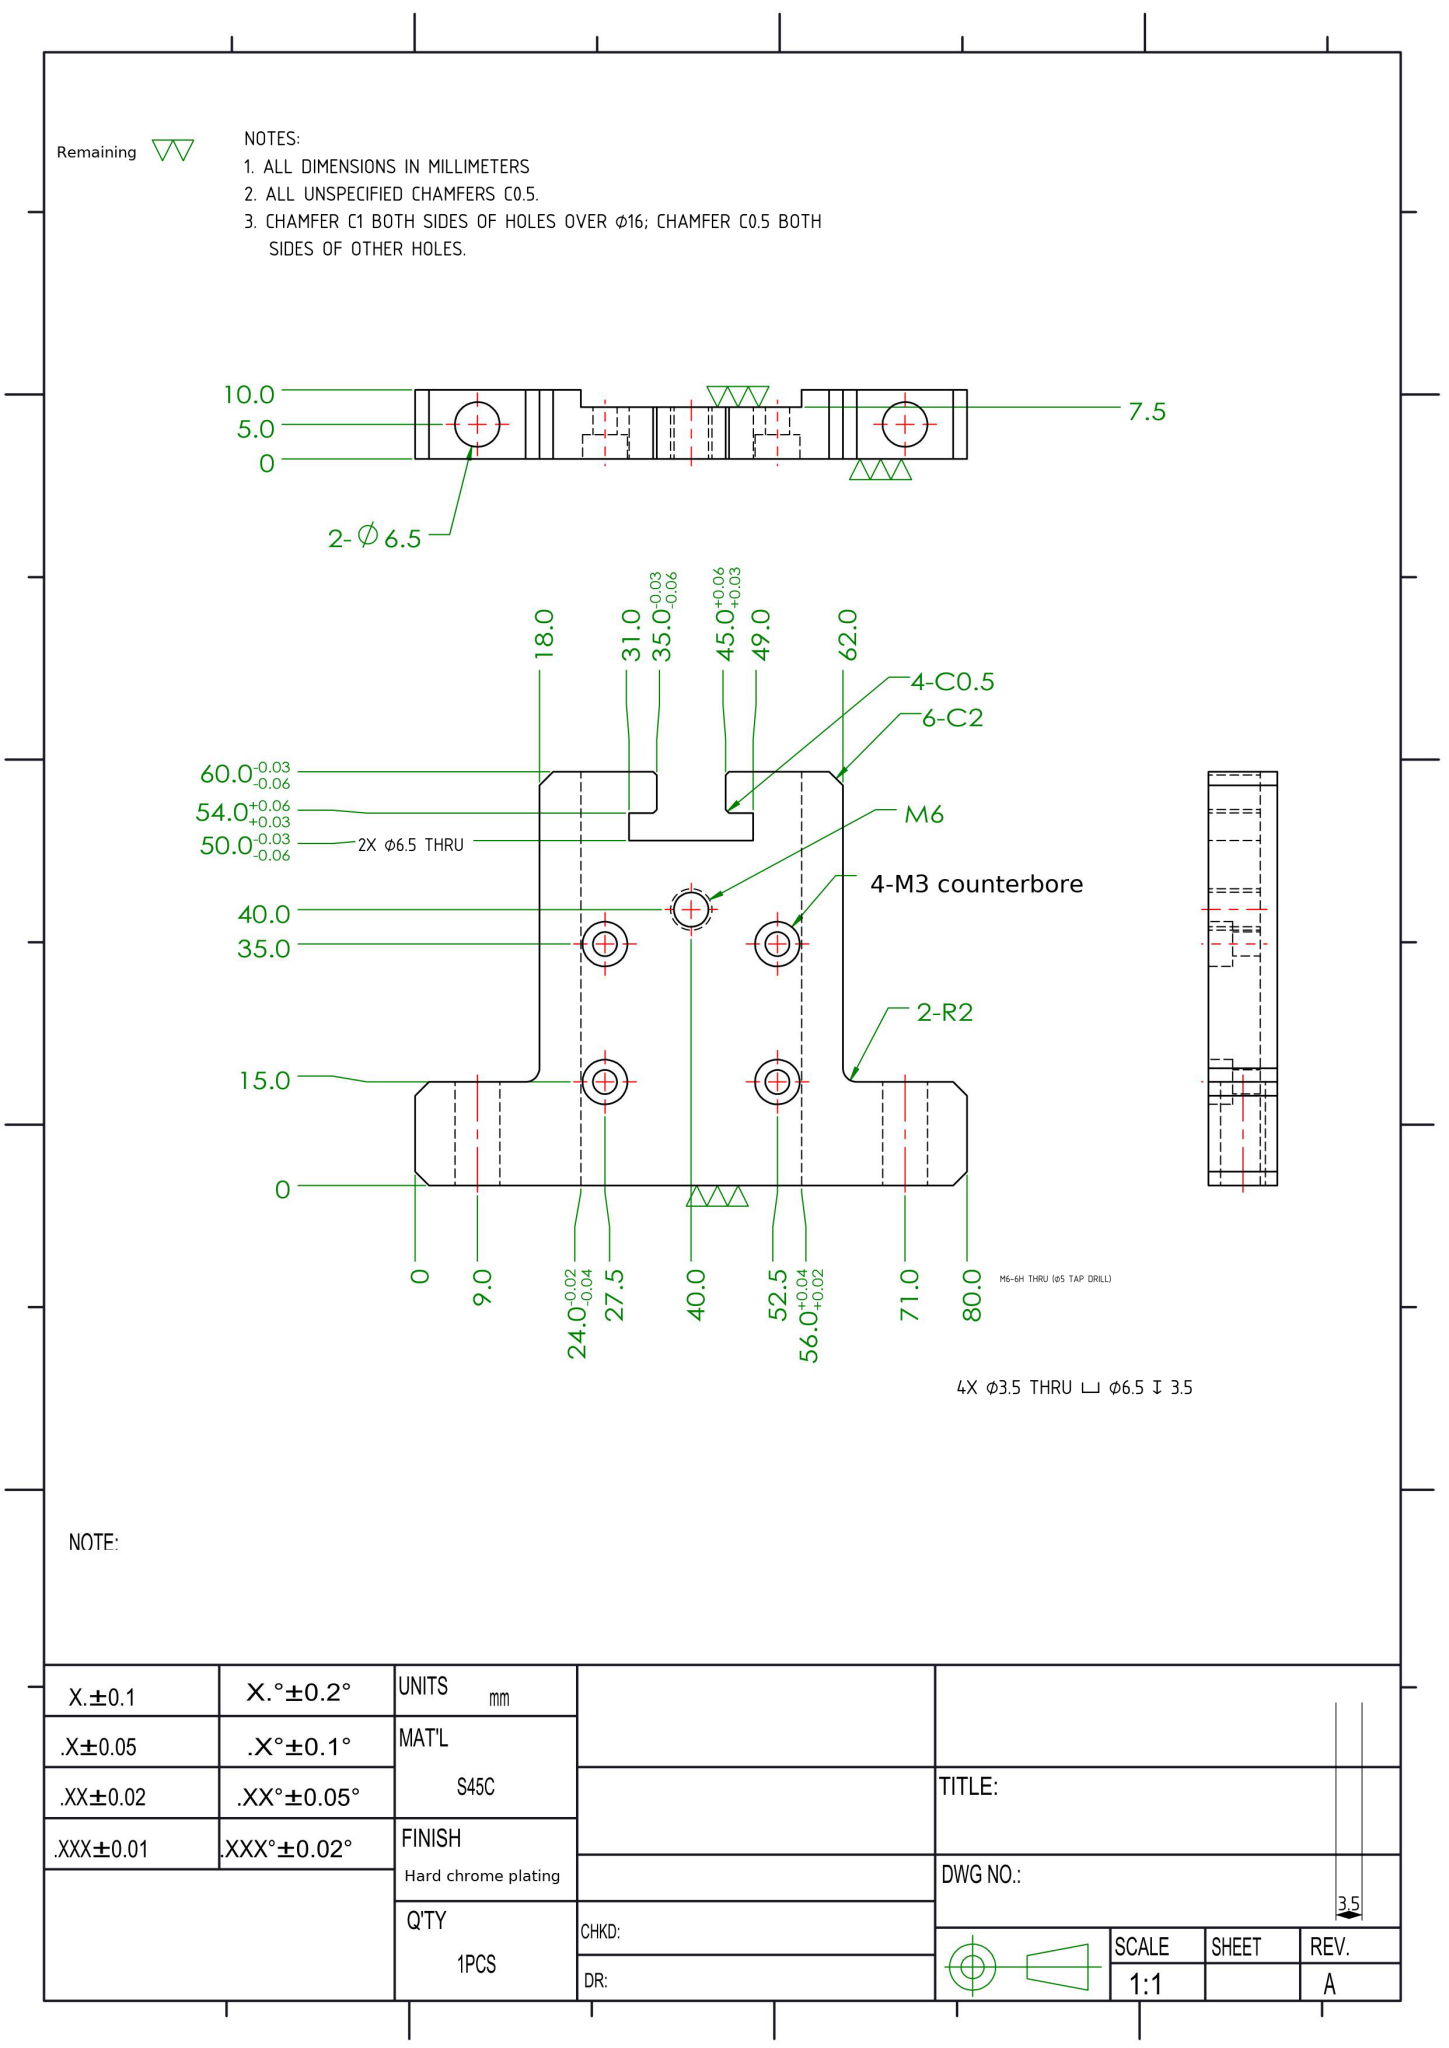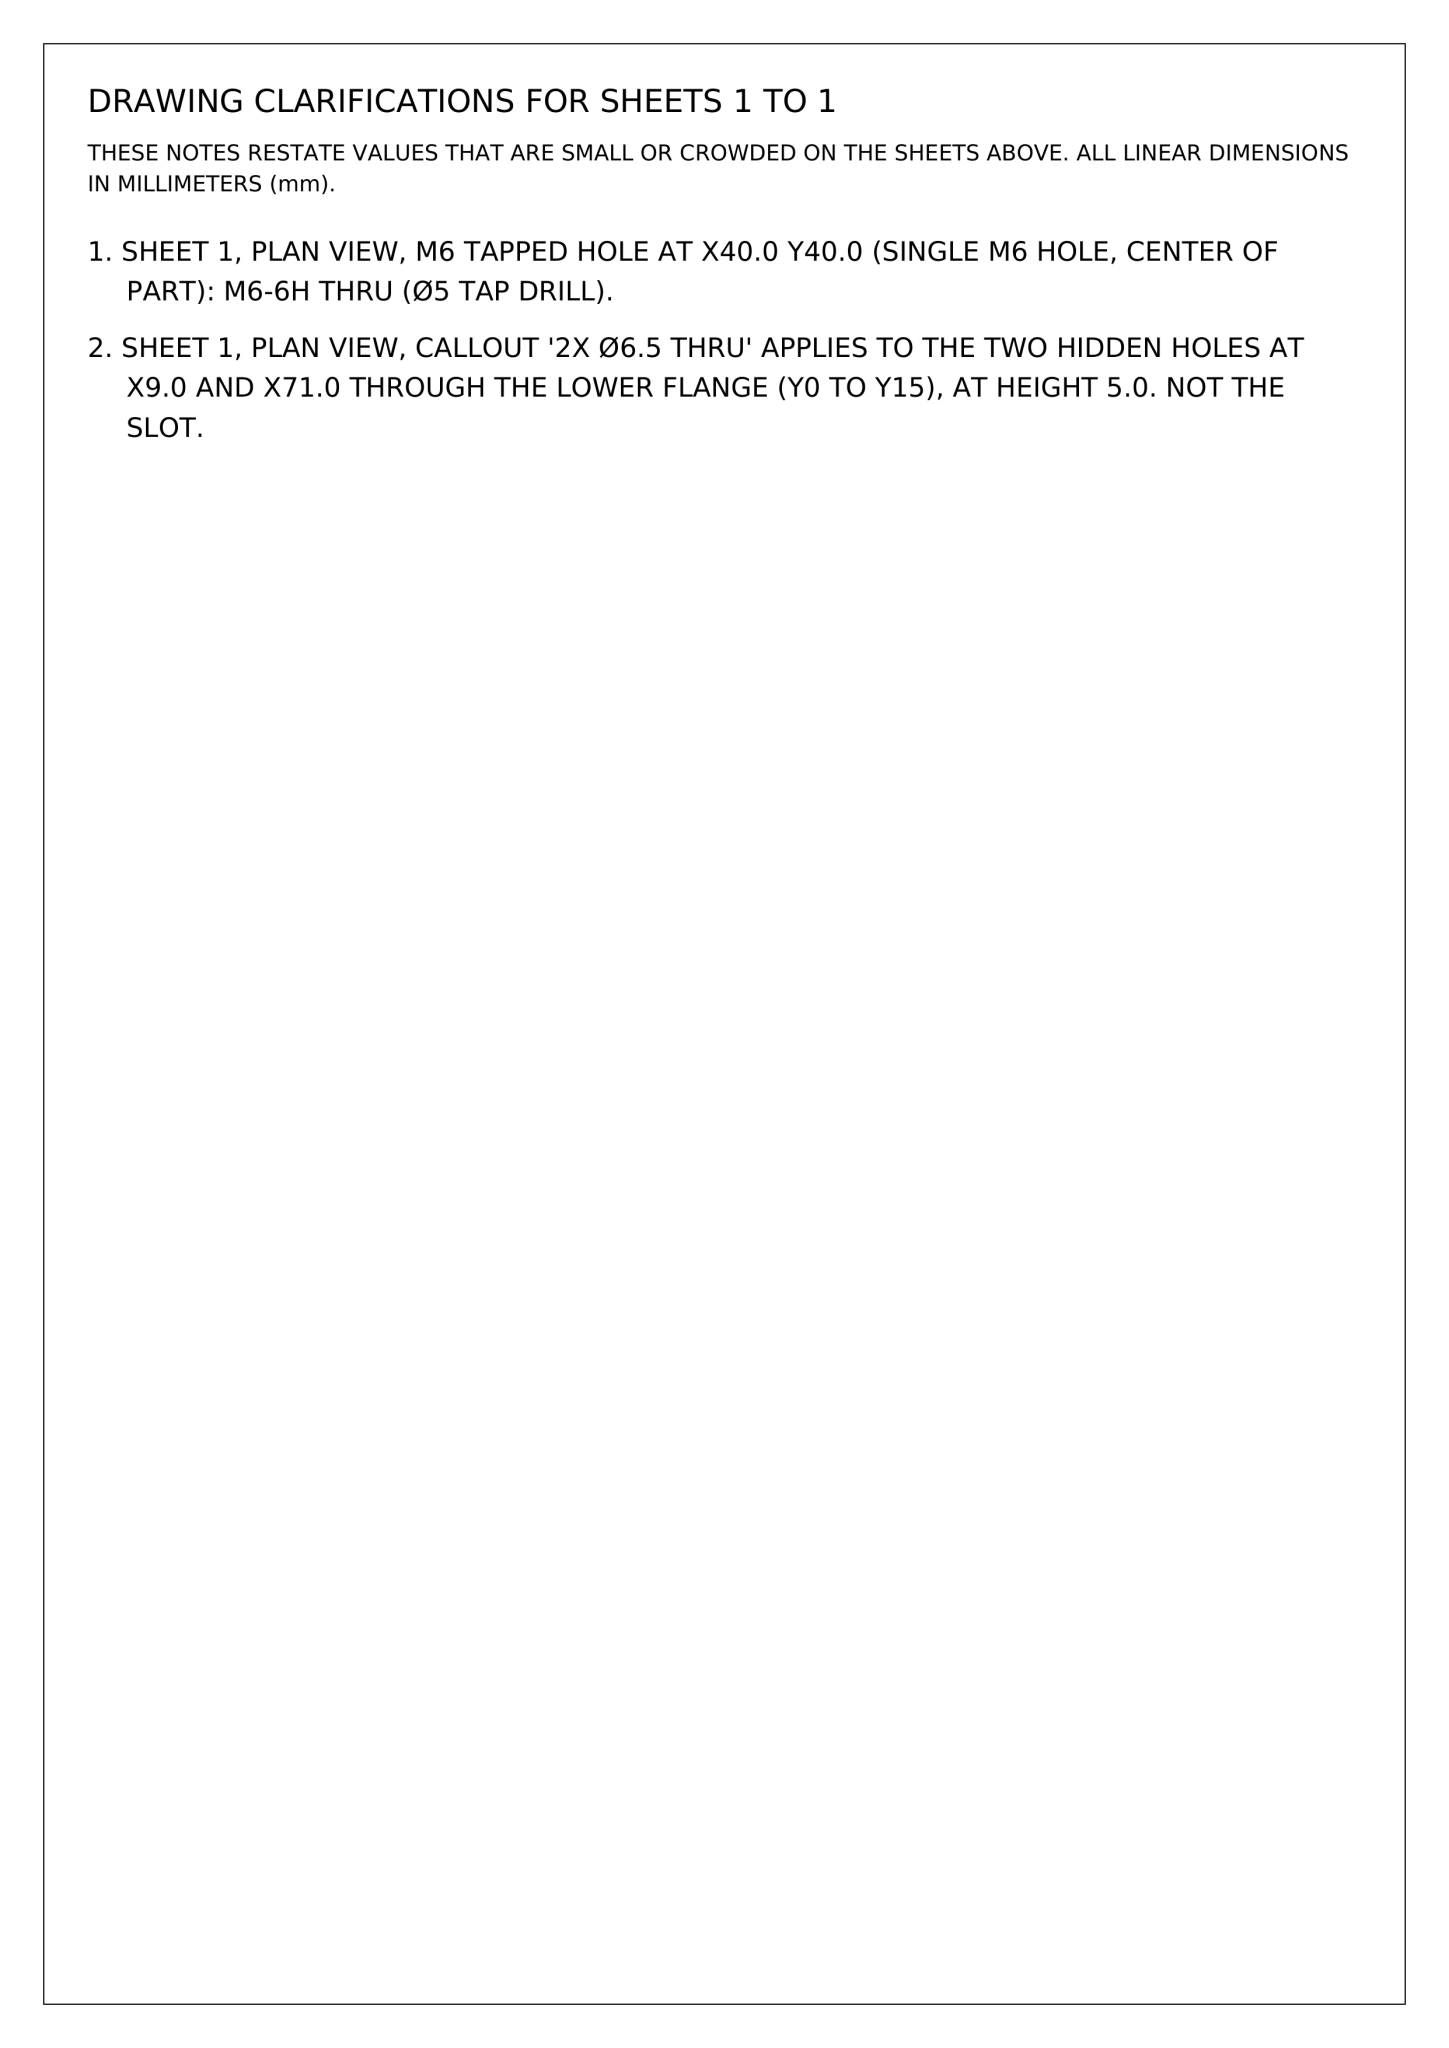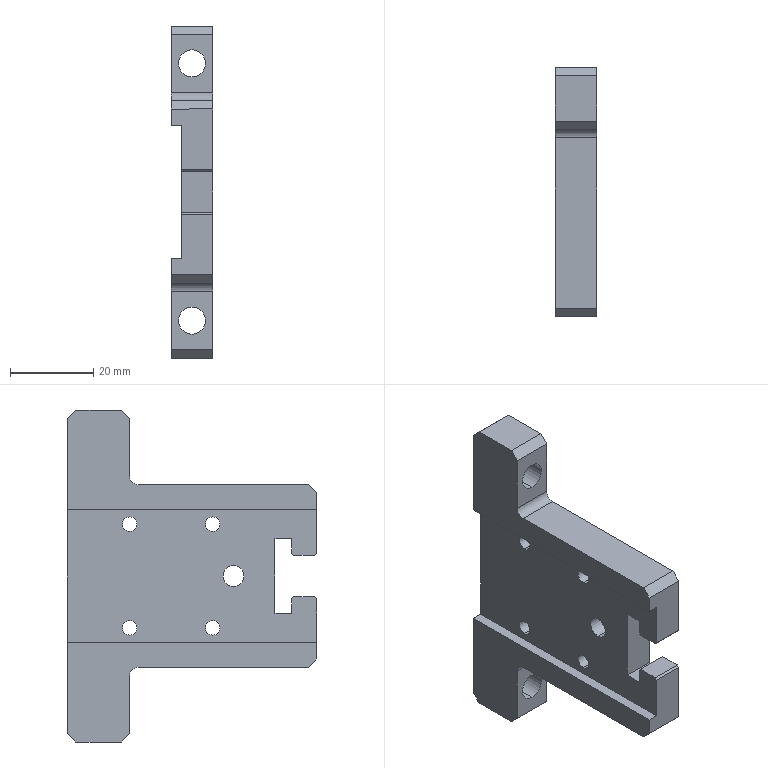Part | NX | mm | 1 solid | 60 faces | box 10 x 60 x 80 mm | volume 24142 mm3 | plane 36 | cylinder 24 | commonest cylinder face diameters 6.5 x12 3.5 x8 5 x2 4 x2